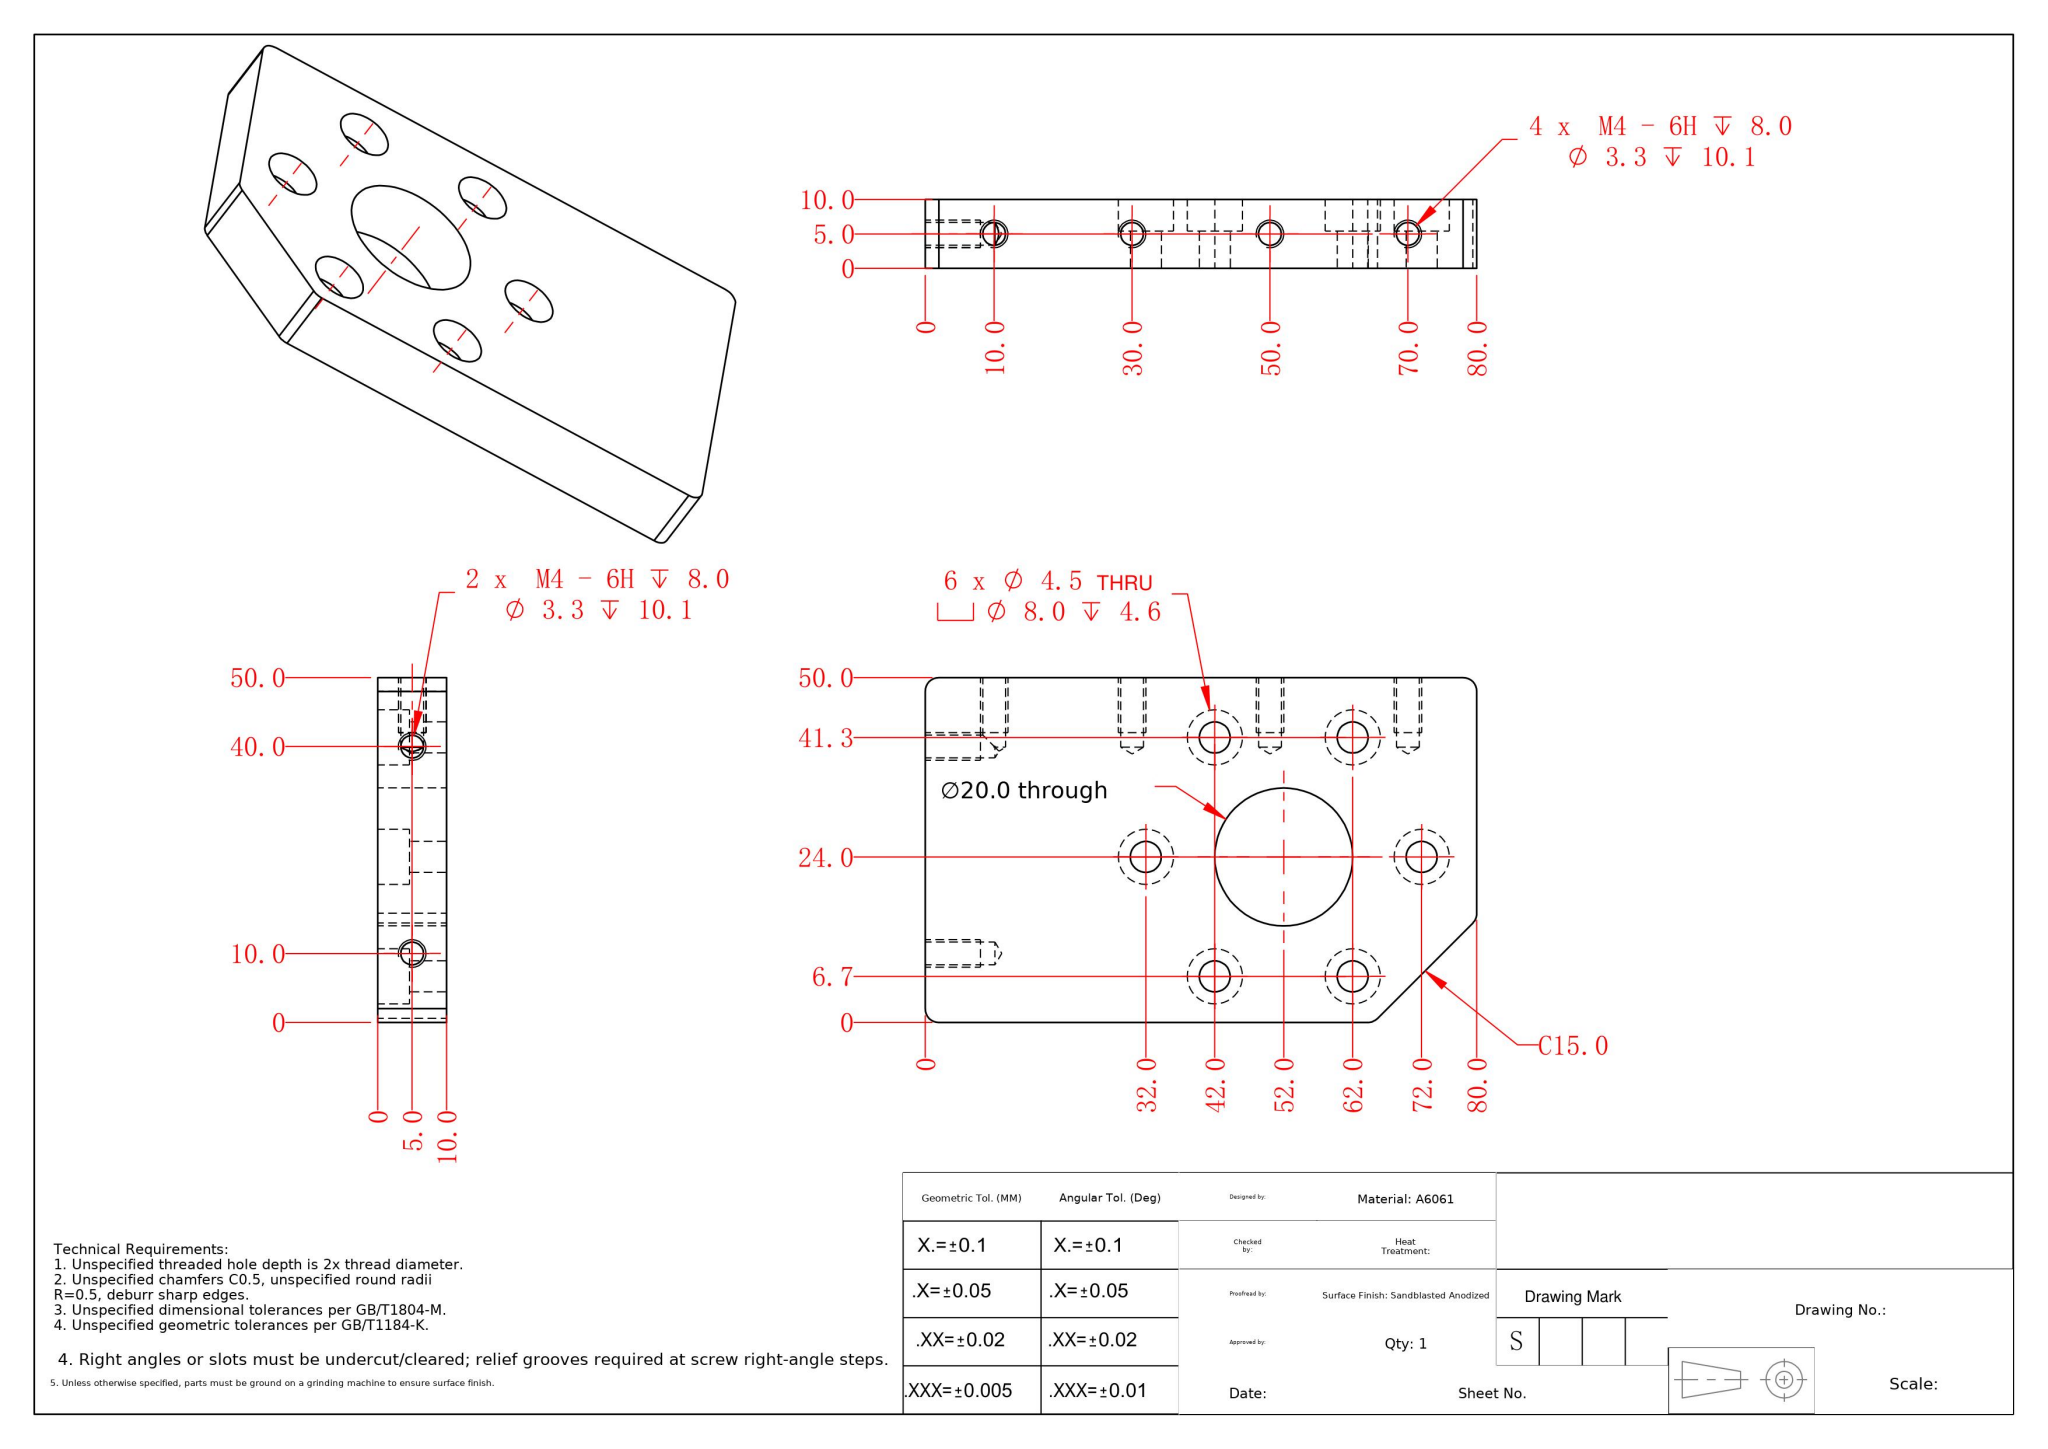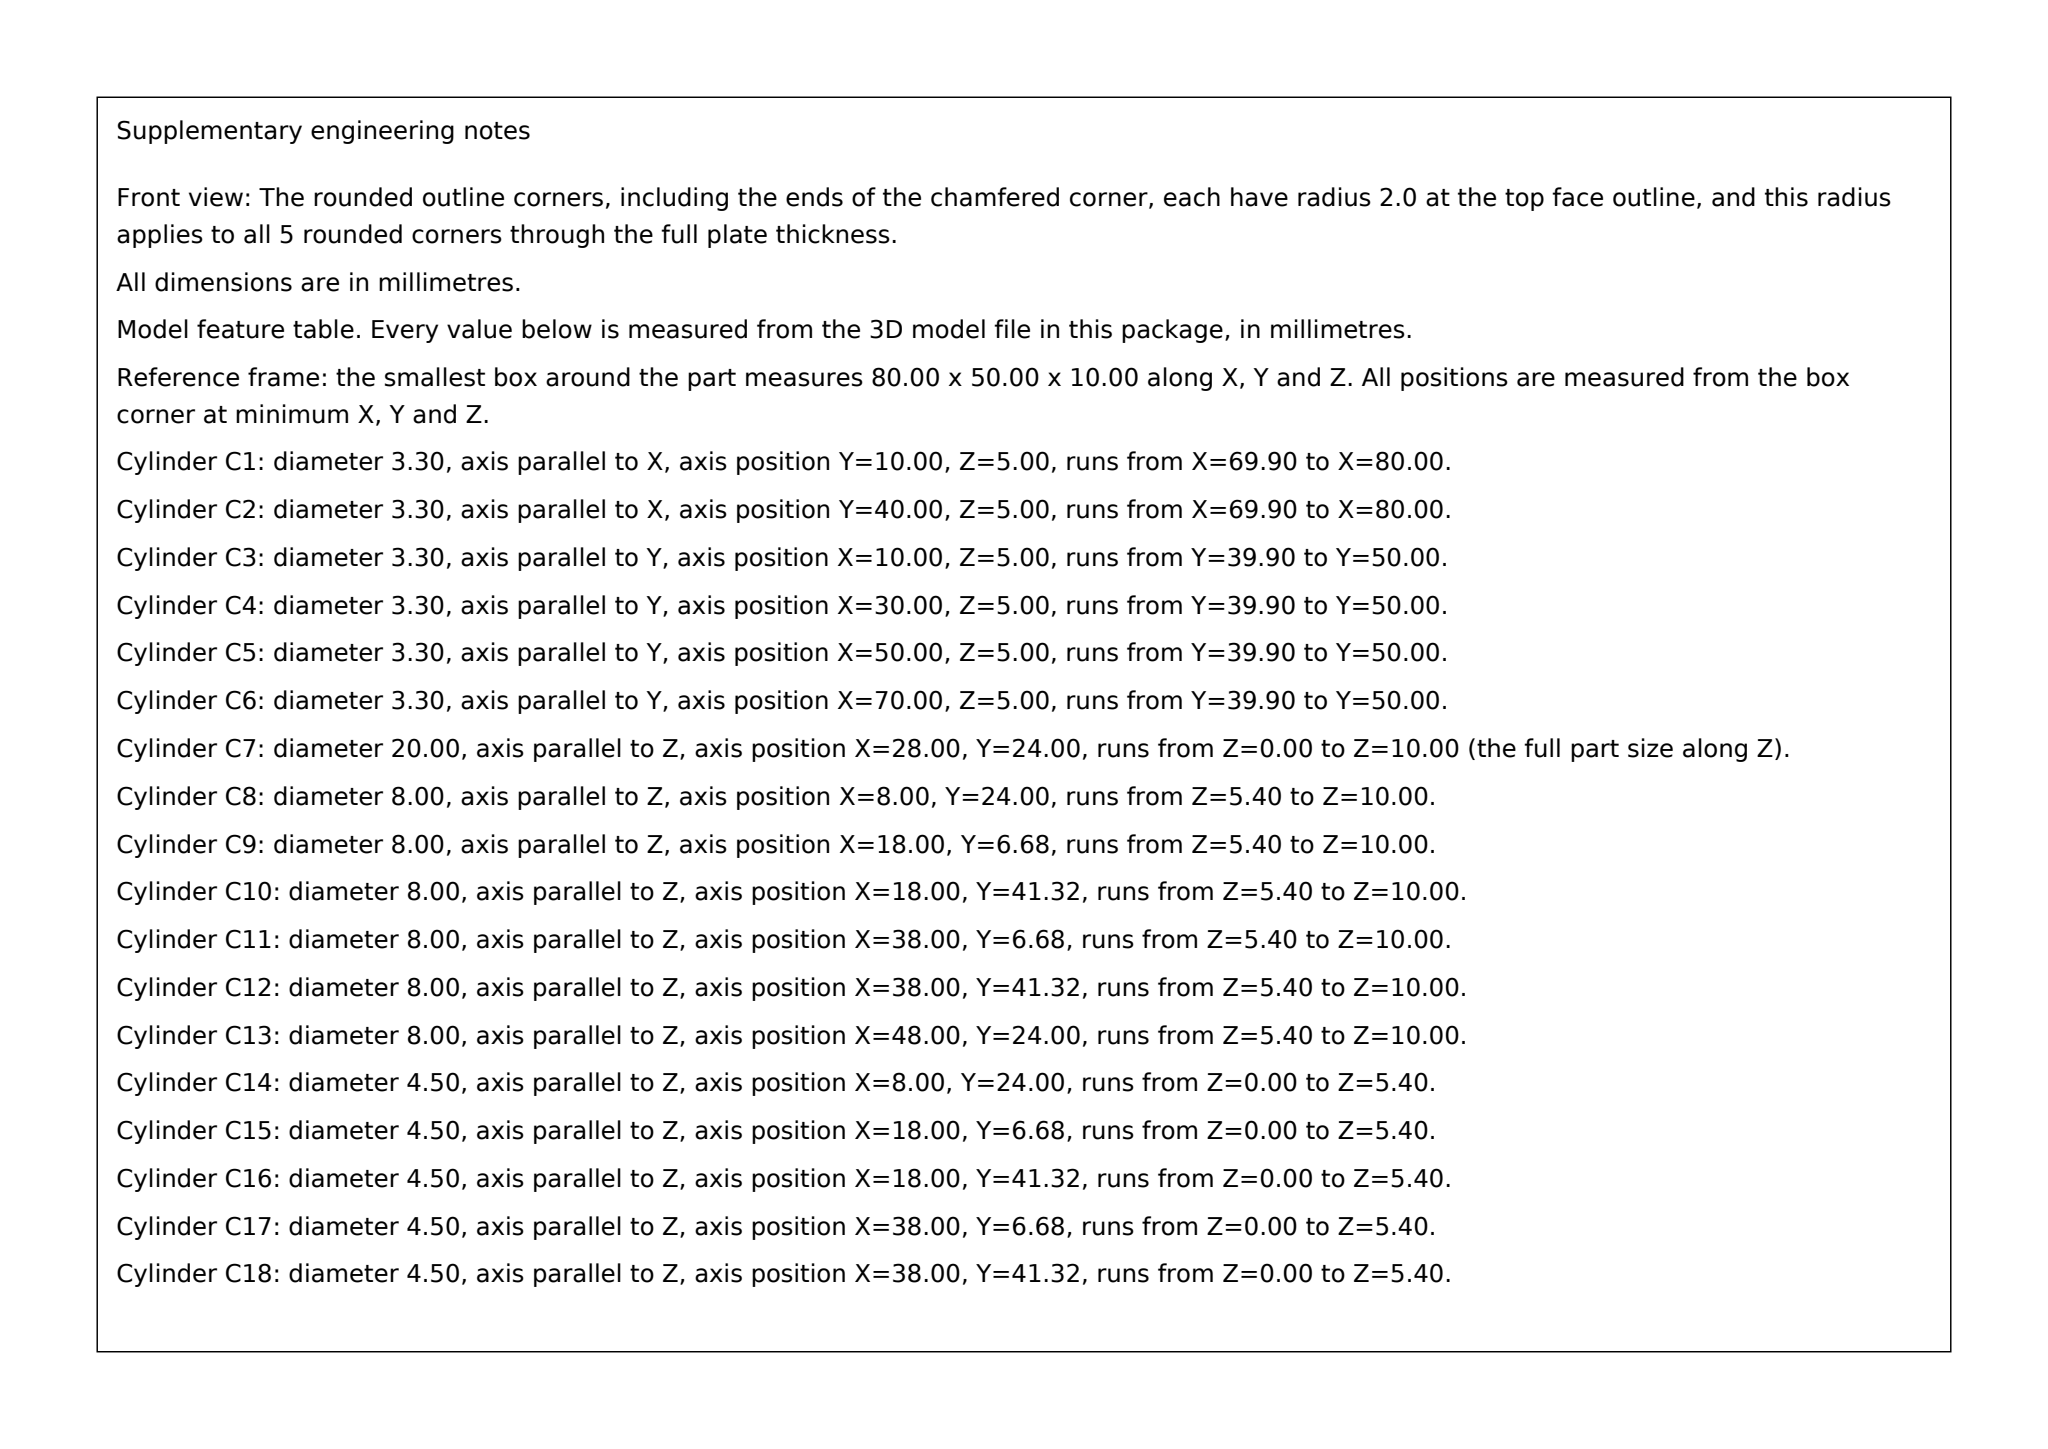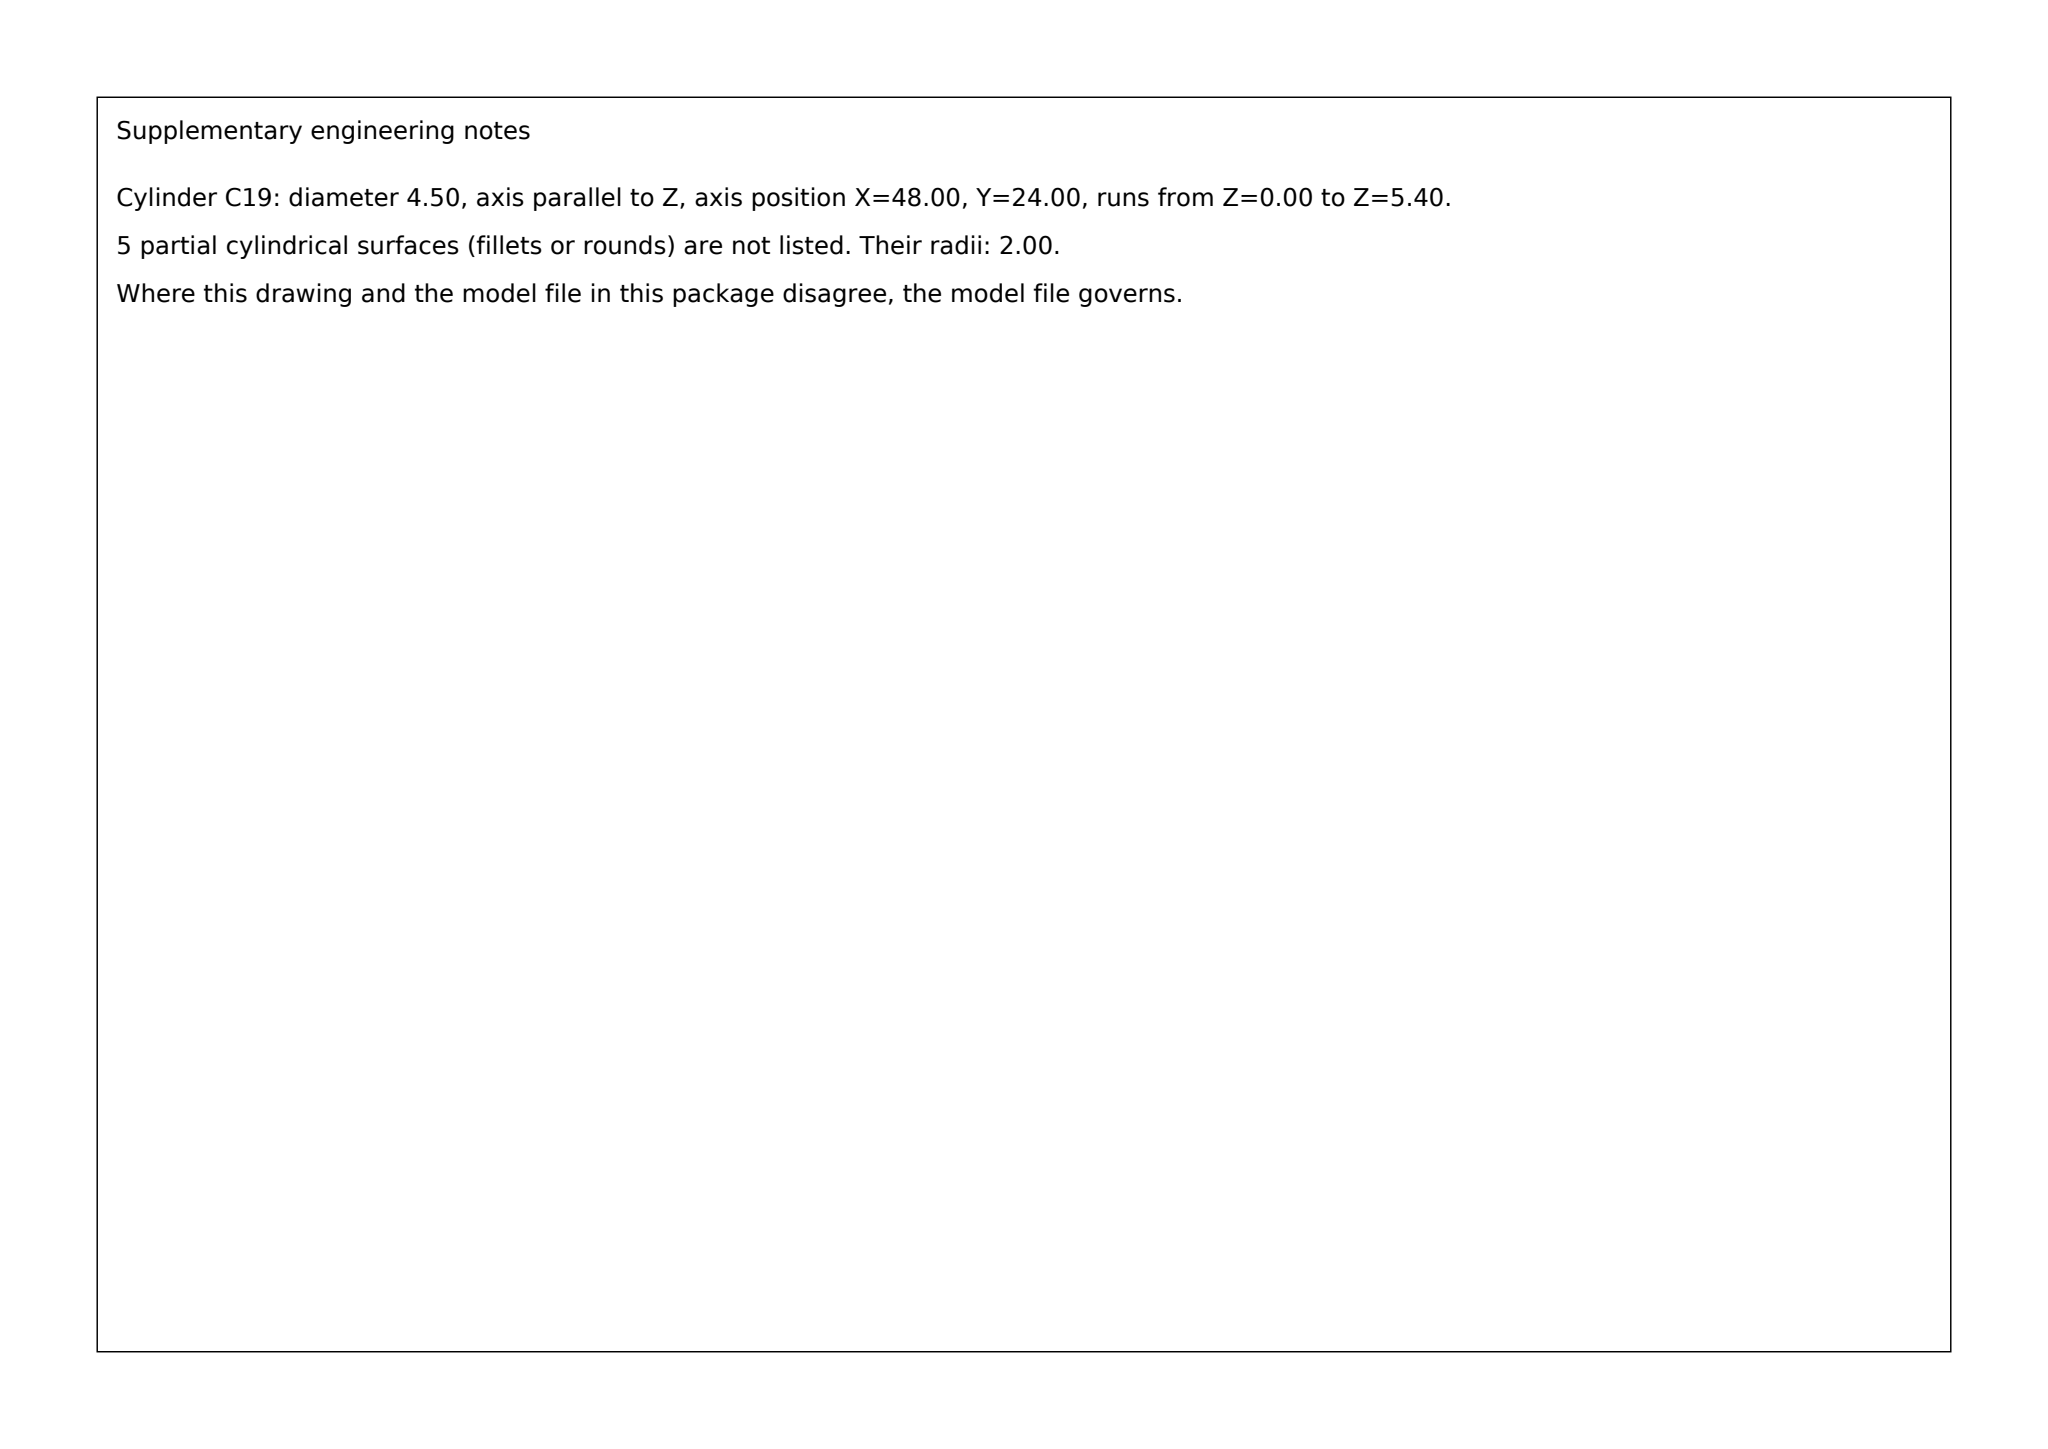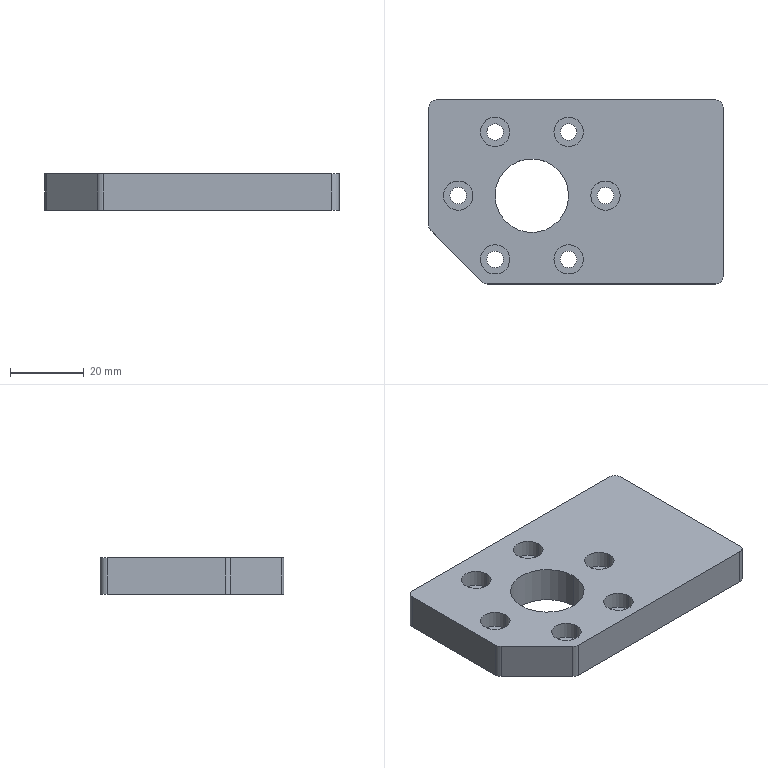Part | SolidWorks | mm | material A6061 | 1 solid | 72 faces | box 80 x 50 x 10 mm | volume 33279 mm3 | cylinder 49 | plane 13 | cone 10 | commonest cylinder face diameters 3.3 x18 8 x12 4.5 x12 4 x5 20 x2
Drawing notes:
5X R2.0 CORNER RADII (QTY 5) - DISREGARD STRAY "11" | from the solid: Five convex arcs dia 4.0 (R2.0) about z at (15.8,2.0),(2.0,15.8),(2.0,48.0),(78.0,2.0),(78.0,48.0), full height 0-10